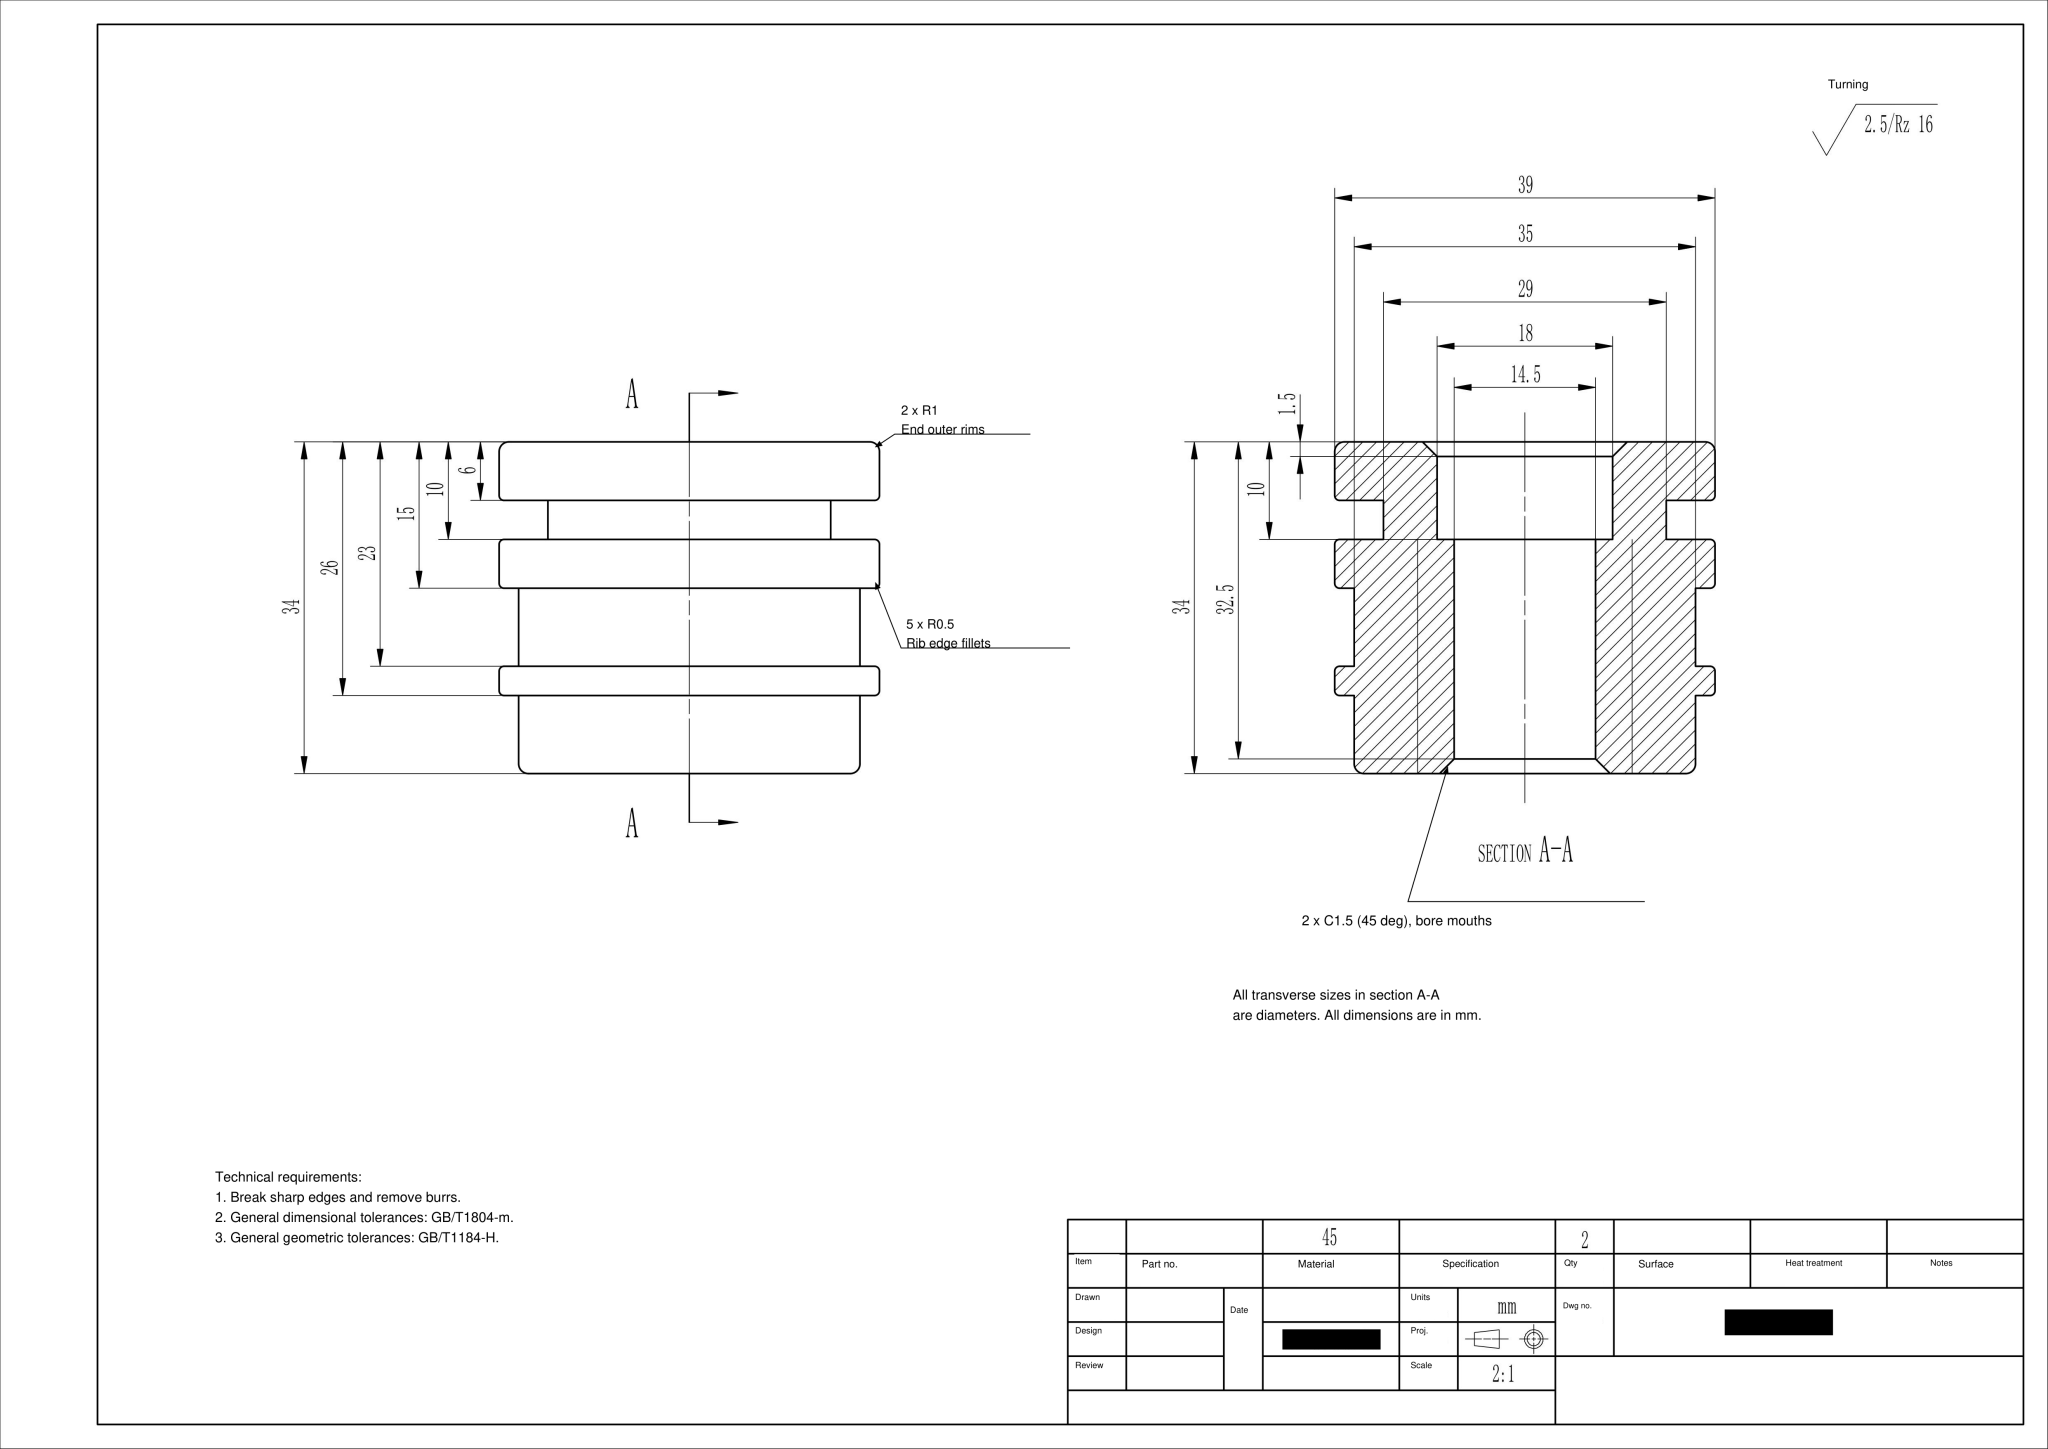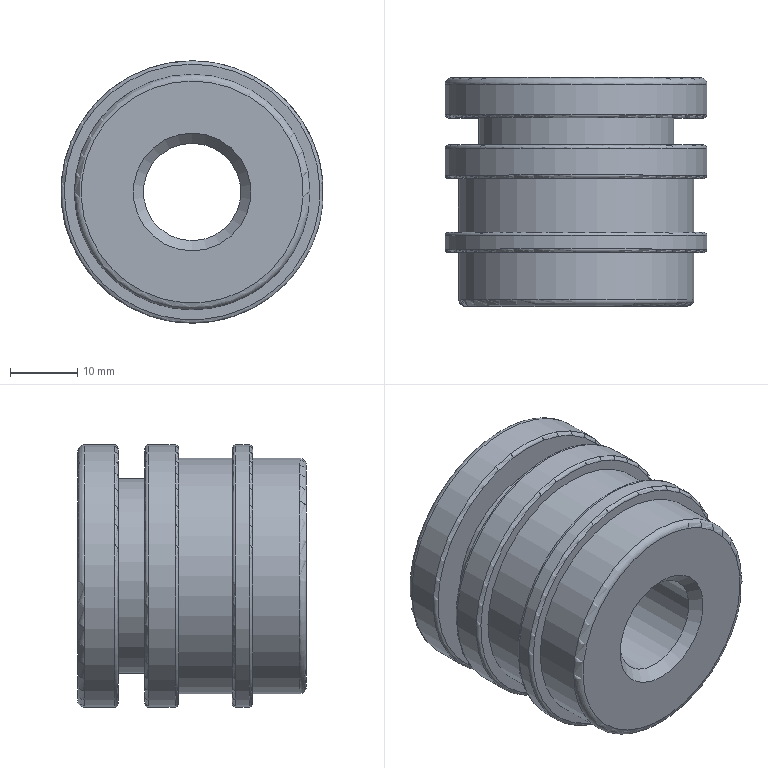Part | NX | mm | 1 solid | 25 faces | box 39 x 34 x 39 mm | volume 28048 mm3 | plane 8 | cylinder 8 | torus 7 | cone 2 | commonest cylinder face diameters 39 x3 35 x2 14.5 x1 18 x1 29 x1
STEP:
#1=CARTESIAN_POINT('',(0.,0.,0.));
#2=DIRECTION('',(0.,0.,1.));
#3=DIRECTION('',(1.,0.,0.));
#4=AXIS2_PLACEMENT_3D('',#1,#2,#3);
#5=(LENGTH_UNIT()NAMED_UNIT(*)SI_UNIT(.MILLI.,.METRE.));
#6=UNCERTAINTY_MEASURE_WITH_UNIT(LENGTH_MEASURE(0.00002),#5,'','');
#7=(NAMED_UNIT(*)PLANE_ANGLE_UNIT()SI_UNIT($,.RADIAN.));
#8=PLANE_ANGLE_MEASURE_WITH_UNIT(PLANE_ANGLE_MEASURE(0.01745),#7);
#9=DIMENSIONAL_EXPONENTS(0.,0.,0.,0.,0.,0.,0.);
#10=(CONVERSION_BASED_UNIT('',#8)NAMED_UNIT(#9)PLANE_ANGLE_UNIT());
#11=(NAMED_UNIT(*)SI_UNIT($,.STERADIAN.)SOLID_ANGLE_UNIT());
#12=(GEOMETRIC_REPRESENTATION_CONTEXT(3)GLOBAL_UNCERTAINTY_ASSIGNED_CONTEXT((#6))GLOBAL_UNIT_ASSIGNED_CONTEXT((#5,#10,#11))REPRESENTATION_CONTEXT('',''));
#13=SHAPE_REPRESENTATION('',(#4),#12);
#14=CARTESIAN_POINT('',(0.,-34.,8.75));
#15=VERTEX_POINT('',#14);
#16=CARTESIAN_POINT('',(0.,-34.,0.));
#17=DIRECTION('',(0.,1.,0.));
#18=DIRECTION('',(0.,0.,1.));
#19=AXIS2_PLACEMENT_3D('',#16,#17,#18);
#20=CIRCLE('',#19,8.75);
#21=EDGE_CURVE('',#15,#15,#20,.T.);
#22=ORIENTED_EDGE('',*,*,#21,.T.);
#23=EDGE_LOOP('',(#22));
#24=FACE_BOUND('',#23,.T.);
#25=CARTESIAN_POINT('',(0.,-34.,16.5));
#26=VERTEX_POINT('',#25);
#27=CARTESIAN_POINT('',(0.,-34.,0.));
#28=DIRECTION('',(0.,-1.,0.));
#29=DIRECTION('',(0.,0.,1.));
#30=AXIS2_PLACEMENT_3D('',#27,#28,#29);
#31=CIRCLE('',#30,16.5);
#32=EDGE_CURVE('',#26,#26,#31,.T.);
#33=ORIENTED_EDGE('',*,*,#32,.T.);
#34=EDGE_LOOP('',(#33));
#35=FACE_BOUND('',#34,.T.);
#36=CARTESIAN_POINT('',(0.,-34.,17.5));
#37=DIRECTION('',(0.,1.,0.));
#38=DIRECTION('',(0.,0.,1.));
#39=AXIS2_PLACEMENT_3D('',#36,#37,#38);
#40=PLANE('',#39);
#41=ADVANCED_FACE('',(#24,#35),#40,.F.);
#42=CARTESIAN_POINT('',(0.,-32.5,7.25));
#43=VERTEX_POINT('',#42);
#44=CARTESIAN_POINT('',(0.,-32.5,0.));
#45=DIRECTION('',(0.,-1.,0.));
#46=DIRECTION('',(0.,0.,1.));
#47=AXIS2_PLACEMENT_3D('',#44,#45,#46);
#48=CIRCLE('',#47,7.25);
#49=EDGE_CURVE('',#43,#43,#48,.T.);
#50=ORIENTED_EDGE('',*,*,#49,.T.);
#51=EDGE_LOOP('',(#50));
#52=FACE_BOUND('',#51,.T.);
#53=CARTESIAN_POINT('',(0.,-10.,-7.25));
#54=VERTEX_POINT('',#53);
#55=CARTESIAN_POINT('',(0.,-10.,0.));
#56=DIRECTION('',(0.,-1.,0.));
#57=DIRECTION('',(0.,0.,-1.));
#58=AXIS2_PLACEMENT_3D('',#55,#56,#57);
#59=CIRCLE('',#58,7.25);
#60=EDGE_CURVE('',#54,#54,#59,.T.);
#61=ORIENTED_EDGE('',*,*,#60,.F.);
#62=EDGE_LOOP('',(#61));
#63=FACE_BOUND('',#62,.T.);
#64=CARTESIAN_POINT('',(0.,0.,0.));
#65=DIRECTION('',(0.,-1.,0.));
#66=DIRECTION('',(0.,0.,-1.));
#67=AXIS2_PLACEMENT_3D('',#64,#65,#66);
#68=CYLINDRICAL_SURFACE('',#67,7.25);
#69=ADVANCED_FACE('',(#52,#63),#68,.F.);
#70=CARTESIAN_POINT('',(0.,-10.,-9.));
#71=VERTEX_POINT('',#70);
#72=CARTESIAN_POINT('',(0.,-10.,0.));
#73=DIRECTION('',(0.,-1.,0.));
#74=DIRECTION('',(0.,0.,-1.));
#75=AXIS2_PLACEMENT_3D('',#72,#73,#74);
#76=CIRCLE('',#75,9.);
#77=EDGE_CURVE('',#71,#71,#76,.T.);
#78=ORIENTED_EDGE('',*,*,#77,.F.);
#79=EDGE_LOOP('',(#78));
#80=FACE_BOUND('',#79,.T.);
#81=ORIENTED_EDGE('',*,*,#60,.T.);
#82=EDGE_LOOP('',(#81));
#83=FACE_BOUND('',#82,.T.);
#84=CARTESIAN_POINT('',(0.,-10.,7.25));
#85=DIRECTION('',(0.,-1.,0.));
#86=DIRECTION('',(0.,0.,-1.));
#87=AXIS2_PLACEMENT_3D('',#84,#85,#86);
#88=PLANE('',#87);
#89=ADVANCED_FACE('',(#80,#83),#88,.F.);
#90=CARTESIAN_POINT('',(0.,-1.5,-9.));
#91=VERTEX_POINT('',#90);
#92=CARTESIAN_POINT('',(0.,-1.5,0.));
#93=DIRECTION('',(0.,1.,0.));
#94=DIRECTION('',(0.,0.,-1.));
#95=AXIS2_PLACEMENT_3D('',#92,#93,#94);
#96=CIRCLE('',#95,9.);
#97=EDGE_CURVE('',#91,#91,#96,.T.);
#98=ORIENTED_EDGE('',*,*,#97,.T.);
#99=EDGE_LOOP('',(#98));
#100=FACE_BOUND('',#99,.T.);
#101=ORIENTED_EDGE('',*,*,#77,.T.);
#102=EDGE_LOOP('',(#101));
#103=FACE_BOUND('',#102,.T.);
#104=CARTESIAN_POINT('',(0.,0.,0.));
#105=DIRECTION('',(0.,-1.,0.));
#106=DIRECTION('',(0.,0.,-1.));
#107=AXIS2_PLACEMENT_3D('',#104,#105,#106);
#108=CYLINDRICAL_SURFACE('',#107,9.);
#109=ADVANCED_FACE('',(#100,#103),#108,.F.);
#110=CARTESIAN_POINT('',(0.,0.,-10.5));
#111=VERTEX_POINT('',#110);
#112=CARTESIAN_POINT('',(0.,0.,0.));
#113=DIRECTION('',(0.,-1.,0.));
#114=DIRECTION('',(0.,0.,-1.));
#115=AXIS2_PLACEMENT_3D('',#112,#113,#114);
#116=CIRCLE('',#115,10.5);
#117=EDGE_CURVE('',#111,#111,#116,.T.);
#118=ORIENTED_EDGE('',*,*,#117,.T.);
#119=EDGE_LOOP('',(#118));
#120=FACE_BOUND('',#119,.T.);
#121=CARTESIAN_POINT('',(0.,0.,-18.5));
#122=VERTEX_POINT('',#121);
#123=CARTESIAN_POINT('',(0.,0.,0.));
#124=DIRECTION('',(0.,1.,0.));
#125=DIRECTION('',(0.,0.,-1.));
#126=AXIS2_PLACEMENT_3D('',#123,#124,#125);
#127=CIRCLE('',#126,18.5);
#128=EDGE_CURVE('',#122,#122,#127,.T.);
#129=ORIENTED_EDGE('',*,*,#128,.T.);
#130=EDGE_LOOP('',(#129));
#131=FACE_BOUND('',#130,.T.);
#132=CARTESIAN_POINT('',(0.,0.,9.));
#133=DIRECTION('',(0.,-1.,0.));
#134=DIRECTION('',(0.,0.,-1.));
#135=AXIS2_PLACEMENT_3D('',#132,#133,#134);
#136=PLANE('',#135);
#137=ADVANCED_FACE('',(#120,#131),#136,.F.);
#138=CARTESIAN_POINT('',(0.,-5.5,19.5));
#139=VERTEX_POINT('',#138);
#140=CARTESIAN_POINT('',(0.,-5.5,0.));
#141=DIRECTION('',(0.,1.,0.));
#142=DIRECTION('',(0.,0.,1.));
#143=AXIS2_PLACEMENT_3D('',#140,#141,#142);
#144=CIRCLE('',#143,19.5);
#145=EDGE_CURVE('',#139,#139,#144,.T.);
#146=ORIENTED_EDGE('',*,*,#145,.T.);
#147=EDGE_LOOP('',(#146));
#148=FACE_BOUND('',#147,.T.);
#149=CARTESIAN_POINT('',(0.,-1.,-19.5));
#150=VERTEX_POINT('',#149);
#151=CARTESIAN_POINT('',(0.,-1.,0.));
#152=DIRECTION('',(0.,-1.,0.));
#153=DIRECTION('',(0.,0.,-1.));
#154=AXIS2_PLACEMENT_3D('',#151,#152,#153);
#155=CIRCLE('',#154,19.5);
#156=EDGE_CURVE('',#150,#150,#155,.T.);
#157=ORIENTED_EDGE('',*,*,#156,.T.);
#158=EDGE_LOOP('',(#157));
#159=FACE_BOUND('',#158,.T.);
#160=CARTESIAN_POINT('',(0.,0.,0.));
#161=DIRECTION('',(0.,-1.,0.));
#162=DIRECTION('',(0.,0.,-1.));
#163=AXIS2_PLACEMENT_3D('',#160,#161,#162);
#164=CYLINDRICAL_SURFACE('',#163,19.5);
#165=ADVANCED_FACE('',(#148,#159),#164,.T.);
#166=CARTESIAN_POINT('',(0.,-6.,19.));
#167=VERTEX_POINT('',#166);
#168=CARTESIAN_POINT('',(0.,-6.,0.));
#169=DIRECTION('',(0.,-1.,0.));
#170=DIRECTION('',(0.,0.,1.));
#171=AXIS2_PLACEMENT_3D('',#168,#169,#170);
#172=CIRCLE('',#171,19.);
#173=EDGE_CURVE('',#167,#167,#172,.T.);
#174=ORIENTED_EDGE('',*,*,#173,.T.);
#175=EDGE_LOOP('',(#174));
#176=FACE_BOUND('',#175,.T.);
#177=CARTESIAN_POINT('',(0.,-6.,-14.5));
#178=VERTEX_POINT('',#177);
#179=CARTESIAN_POINT('',(0.,-6.,0.));
#180=DIRECTION('',(0.,-1.,0.));
#181=DIRECTION('',(0.,0.,-1.));
#182=AXIS2_PLACEMENT_3D('',#179,#180,#181);
#183=CIRCLE('',#182,14.5);
#184=EDGE_CURVE('',#178,#178,#183,.T.);
#185=ORIENTED_EDGE('',*,*,#184,.F.);
#186=EDGE_LOOP('',(#185));
#187=FACE_BOUND('',#186,.T.);
#188=CARTESIAN_POINT('',(0.,-6.,19.5));
#189=DIRECTION('',(0.,1.,0.));
#190=DIRECTION('',(0.,0.,1.));
#191=AXIS2_PLACEMENT_3D('',#188,#189,#190);
#192=PLANE('',#191);
#193=ADVANCED_FACE('',(#176,#187),#192,.F.);
#194=CARTESIAN_POINT('',(0.,-10.,-14.5));
#195=VERTEX_POINT('',#194);
#196=CARTESIAN_POINT('',(0.,-10.,0.));
#197=DIRECTION('',(0.,-1.,0.));
#198=DIRECTION('',(0.,0.,-1.));
#199=AXIS2_PLACEMENT_3D('',#196,#197,#198);
#200=CIRCLE('',#199,14.5);
#201=EDGE_CURVE('',#195,#195,#200,.T.);
#202=ORIENTED_EDGE('',*,*,#201,.F.);
#203=EDGE_LOOP('',(#202));
#204=FACE_BOUND('',#203,.T.);
#205=ORIENTED_EDGE('',*,*,#184,.T.);
#206=EDGE_LOOP('',(#205));
#207=FACE_BOUND('',#206,.T.);
#208=CARTESIAN_POINT('',(0.,0.,0.));
#209=DIRECTION('',(0.,-1.,0.));
#210=DIRECTION('',(0.,0.,-1.));
#211=AXIS2_PLACEMENT_3D('',#208,#209,#210);
#212=CYLINDRICAL_SURFACE('',#211,14.5);
#213=ADVANCED_FACE('',(#204,#207),#212,.T.);
#214=CARTESIAN_POINT('',(0.,-10.,-19.));
#215=VERTEX_POINT('',#214);
#216=CARTESIAN_POINT('',(0.,-10.,0.));
#217=DIRECTION('',(0.,1.,0.));
#218=DIRECTION('',(0.,0.,-1.));
#219=AXIS2_PLACEMENT_3D('',#216,#217,#218);
#220=CIRCLE('',#219,19.);
#221=EDGE_CURVE('',#215,#215,#220,.T.);
#222=ORIENTED_EDGE('',*,*,#221,.T.);
#223=EDGE_LOOP('',(#222));
#224=FACE_BOUND('',#223,.T.);
#225=ORIENTED_EDGE('',*,*,#201,.T.);
#226=EDGE_LOOP('',(#225));
#227=FACE_BOUND('',#226,.T.);
#228=CARTESIAN_POINT('',(0.,-10.,14.5));
#229=DIRECTION('',(0.,-1.,0.));
#230=DIRECTION('',(0.,0.,-1.));
#231=AXIS2_PLACEMENT_3D('',#228,#229,#230);
#232=PLANE('',#231);
#233=ADVANCED_FACE('',(#224,#227),#232,.F.);
#234=CARTESIAN_POINT('',(0.,-14.5,19.5));
#235=VERTEX_POINT('',#234);
#236=CARTESIAN_POINT('',(0.,-14.5,0.));
#237=DIRECTION('',(0.,1.,0.));
#238=DIRECTION('',(0.,0.,1.));
#239=AXIS2_PLACEMENT_3D('',#236,#237,#238);
#240=CIRCLE('',#239,19.5);
#241=EDGE_CURVE('',#235,#235,#240,.T.);
#242=ORIENTED_EDGE('',*,*,#241,.T.);
#243=EDGE_LOOP('',(#242));
#244=FACE_BOUND('',#243,.T.);
#245=CARTESIAN_POINT('',(0.,-10.5,-19.5));
#246=VERTEX_POINT('',#245);
#247=CARTESIAN_POINT('',(0.,-10.5,0.));
#248=DIRECTION('',(0.,-1.,0.));
#249=DIRECTION('',(0.,0.,-1.));
#250=AXIS2_PLACEMENT_3D('',#247,#248,#249);
#251=CIRCLE('',#250,19.5);
#252=EDGE_CURVE('',#246,#246,#251,.T.);
#253=ORIENTED_EDGE('',*,*,#252,.T.);
#254=EDGE_LOOP('',(#253));
#255=FACE_BOUND('',#254,.T.);
#256=CARTESIAN_POINT('',(0.,0.,0.));
#257=DIRECTION('',(0.,-1.,0.));
#258=DIRECTION('',(0.,0.,-1.));
#259=AXIS2_PLACEMENT_3D('',#256,#257,#258);
#260=CYLINDRICAL_SURFACE('',#259,19.5);
#261=ADVANCED_FACE('',(#244,#255),#260,.T.);
#262=CARTESIAN_POINT('',(0.,-15.,19.));
#263=VERTEX_POINT('',#262);
#264=CARTESIAN_POINT('',(0.,-15.,0.));
#265=DIRECTION('',(0.,-1.,0.));
#266=DIRECTION('',(0.,0.,1.));
#267=AXIS2_PLACEMENT_3D('',#264,#265,#266);
#268=CIRCLE('',#267,19.);
#269=EDGE_CURVE('',#263,#263,#268,.T.);
#270=ORIENTED_EDGE('',*,*,#269,.T.);
#271=EDGE_LOOP('',(#270));
#272=FACE_BOUND('',#271,.T.);
#273=CARTESIAN_POINT('',(0.,-15.,-17.5));
#274=VERTEX_POINT('',#273);
#275=CARTESIAN_POINT('',(0.,-15.,0.));
#276=DIRECTION('',(0.,-1.,0.));
#277=DIRECTION('',(0.,0.,-1.));
#278=AXIS2_PLACEMENT_3D('',#275,#276,#277);
#279=CIRCLE('',#278,17.5);
#280=EDGE_CURVE('',#274,#274,#279,.T.);
#281=ORIENTED_EDGE('',*,*,#280,.F.);
#282=EDGE_LOOP('',(#281));
#283=FACE_BOUND('',#282,.T.);
#284=CARTESIAN_POINT('',(0.,-15.,19.5));
#285=DIRECTION('',(0.,1.,0.));
#286=DIRECTION('',(0.,0.,1.));
#287=AXIS2_PLACEMENT_3D('',#284,#285,#286);
#288=PLANE('',#287);
#289=ADVANCED_FACE('',(#272,#283),#288,.F.);
#290=CARTESIAN_POINT('',(0.,-23.,-17.5));
#291=VERTEX_POINT('',#290);
#292=CARTESIAN_POINT('',(0.,-23.,0.));
#293=DIRECTION('',(0.,-1.,0.));
#294=DIRECTION('',(0.,0.,-1.));
#295=AXIS2_PLACEMENT_3D('',#292,#293,#294);
#296=CIRCLE('',#295,17.5);
#297=EDGE_CURVE('',#291,#291,#296,.T.);
#298=ORIENTED_EDGE('',*,*,#297,.F.);
#299=EDGE_LOOP('',(#298));
#300=FACE_BOUND('',#299,.T.);
#301=ORIENTED_EDGE('',*,*,#280,.T.);
#302=EDGE_LOOP('',(#301));
#303=FACE_BOUND('',#302,.T.);
#304=CARTESIAN_POINT('',(0.,0.,0.));
#305=DIRECTION('',(0.,-1.,0.));
#306=DIRECTION('',(0.,0.,-1.));
#307=AXIS2_PLACEMENT_3D('',#304,#305,#306);
#308=CYLINDRICAL_SURFACE('',#307,17.5);
#309=ADVANCED_FACE('',(#300,#303),#308,.T.);
#310=CARTESIAN_POINT('',(0.,-23.,-19.));
#311=VERTEX_POINT('',#310);
#312=CARTESIAN_POINT('',(0.,-23.,0.));
#313=DIRECTION('',(0.,1.,0.));
#314=DIRECTION('',(0.,0.,-1.));
#315=AXIS2_PLACEMENT_3D('',#312,#313,#314);
#316=CIRCLE('',#315,19.);
#317=EDGE_CURVE('',#311,#311,#316,.T.);
#318=ORIENTED_EDGE('',*,*,#317,.T.);
#319=EDGE_LOOP('',(#318));
#320=FACE_BOUND('',#319,.T.);
#321=ORIENTED_EDGE('',*,*,#297,.T.);
#322=EDGE_LOOP('',(#321));
#323=FACE_BOUND('',#322,.T.);
#324=CARTESIAN_POINT('',(0.,-23.,17.5));
#325=DIRECTION('',(0.,-1.,0.));
#326=DIRECTION('',(0.,0.,-1.));
#327=AXIS2_PLACEMENT_3D('',#324,#325,#326);
#328=PLANE('',#327);
#329=ADVANCED_FACE('',(#320,#323),#328,.F.);
#330=CARTESIAN_POINT('',(0.,-25.5,19.5));
#331=VERTEX_POINT('',#330);
#332=CARTESIAN_POINT('',(0.,-25.5,0.));
#333=DIRECTION('',(0.,1.,0.));
#334=DIRECTION('',(0.,0.,1.));
#335=AXIS2_PLACEMENT_3D('',#332,#333,#334);
#336=CIRCLE('',#335,19.5);
#337=EDGE_CURVE('',#331,#331,#336,.T.);
#338=ORIENTED_EDGE('',*,*,#337,.T.);
#339=EDGE_LOOP('',(#338));
#340=FACE_BOUND('',#339,.T.);
#341=CARTESIAN_POINT('',(0.,-23.5,-19.5));
#342=VERTEX_POINT('',#341);
#343=CARTESIAN_POINT('',(0.,-23.5,0.));
#344=DIRECTION('',(0.,-1.,0.));
#345=DIRECTION('',(0.,0.,-1.));
#346=AXIS2_PLACEMENT_3D('',#343,#344,#345);
#347=CIRCLE('',#346,19.5);
#348=EDGE_CURVE('',#342,#342,#347,.T.);
#349=ORIENTED_EDGE('',*,*,#348,.T.);
#350=EDGE_LOOP('',(#349));
#351=FACE_BOUND('',#350,.T.);
#352=CARTESIAN_POINT('',(0.,0.,0.));
#353=DIRECTION('',(0.,-1.,0.));
#354=DIRECTION('',(0.,0.,-1.));
#355=AXIS2_PLACEMENT_3D('',#352,#353,#354);
#356=CYLINDRICAL_SURFACE('',#355,19.5);
#357=ADVANCED_FACE('',(#340,#351),#356,.T.);
#358=CARTESIAN_POINT('',(0.,-26.,19.));
#359=VERTEX_POINT('',#358);
#360=CARTESIAN_POINT('',(0.,-26.,0.));
#361=DIRECTION('',(0.,-1.,0.));
#362=DIRECTION('',(0.,0.,1.));
#363=AXIS2_PLACEMENT_3D('',#360,#361,#362);
#364=CIRCLE('',#363,19.);
#365=EDGE_CURVE('',#359,#359,#364,.T.);
#366=ORIENTED_EDGE('',*,*,#365,.T.);
#367=EDGE_LOOP('',(#366));
#368=FACE_BOUND('',#367,.T.);
#369=CARTESIAN_POINT('',(0.,-26.,-17.5));
#370=VERTEX_POINT('',#369);
#371=CARTESIAN_POINT('',(0.,-26.,0.));
#372=DIRECTION('',(0.,-1.,0.));
#373=DIRECTION('',(0.,0.,-1.));
#374=AXIS2_PLACEMENT_3D('',#371,#372,#373);
#375=CIRCLE('',#374,17.5);
#376=EDGE_CURVE('',#370,#370,#375,.T.);
#377=ORIENTED_EDGE('',*,*,#376,.F.);
#378=EDGE_LOOP('',(#377));
#379=FACE_BOUND('',#378,.T.);
#380=CARTESIAN_POINT('',(0.,-26.,19.5));
#381=DIRECTION('',(0.,1.,0.));
#382=DIRECTION('',(0.,0.,1.));
#383=AXIS2_PLACEMENT_3D('',#380,#381,#382);
#384=PLANE('',#383);
#385=ADVANCED_FACE('',(#368,#379),#384,.F.);
#386=CARTESIAN_POINT('',(0.,-33.,17.5));
#387=VERTEX_POINT('',#386);
#388=CARTESIAN_POINT('',(0.,-33.,0.));
#389=DIRECTION('',(0.,1.,0.));
#390=DIRECTION('',(0.,0.,1.));
#391=AXIS2_PLACEMENT_3D('',#388,#389,#390);
#392=CIRCLE('',#391,17.5);
#393=EDGE_CURVE('',#387,#387,#392,.T.);
#394=ORIENTED_EDGE('',*,*,#393,.T.);
#395=EDGE_LOOP('',(#394));
#396=FACE_BOUND('',#395,.T.);
#397=ORIENTED_EDGE('',*,*,#376,.T.);
#398=EDGE_LOOP('',(#397));
#399=FACE_BOUND('',#398,.T.);
#400=CARTESIAN_POINT('',(0.,0.,0.));
#401=DIRECTION('',(0.,-1.,0.));
#402=DIRECTION('',(0.,0.,-1.));
#403=AXIS2_PLACEMENT_3D('',#400,#401,#402);
#404=CYLINDRICAL_SURFACE('',#403,17.5);
#405=ADVANCED_FACE('',(#396,#399),#404,.T.);
#406=ORIENTED_EDGE('',*,*,#393,.F.);
#407=EDGE_LOOP('',(#406));
#408=FACE_BOUND('',#407,.T.);
#409=ORIENTED_EDGE('',*,*,#32,.F.);
#410=EDGE_LOOP('',(#409));
#411=FACE_BOUND('',#410,.T.);
#412=CARTESIAN_POINT('',(0.,-33.,0.));
#413=DIRECTION('',(0.,1.,0.));
#414=DIRECTION('',(0.,0.,1.));
#415=AXIS2_PLACEMENT_3D('',#412,#413,#414);
#416=TOROIDAL_SURFACE('',#415,16.5,1.);
#417=ADVANCED_FACE('',(#408,#411),#416,.T.);
#418=ORIENTED_EDGE('',*,*,#128,.F.);
#419=EDGE_LOOP('',(#418));
#420=FACE_BOUND('',#419,.T.);
#421=ORIENTED_EDGE('',*,*,#156,.F.);
#422=EDGE_LOOP('',(#421));
#423=FACE_BOUND('',#422,.T.);
#424=CARTESIAN_POINT('',(0.,-1.,0.));
#425=DIRECTION('',(0.,-1.,0.));
#426=DIRECTION('',(0.,0.,-1.));
#427=AXIS2_PLACEMENT_3D('',#424,#425,#426);
#428=TOROIDAL_SURFACE('',#427,18.5,1.);
#429=ADVANCED_FACE('',(#420,#423),#428,.T.);
#430=ORIENTED_EDGE('',*,*,#337,.F.);
#431=EDGE_LOOP('',(#430));
#432=FACE_BOUND('',#431,.T.);
#433=ORIENTED_EDGE('',*,*,#365,.F.);
#434=EDGE_LOOP('',(#433));
#435=FACE_BOUND('',#434,.T.);
#436=CARTESIAN_POINT('',(0.,-25.5,0.));
#437=DIRECTION('',(0.,1.,0.));
#438=DIRECTION('',(0.,0.,1.));
#439=AXIS2_PLACEMENT_3D('',#436,#437,#438);
#440=TOROIDAL_SURFACE('',#439,19.,0.5);
#441=ADVANCED_FACE('',(#432,#435),#440,.T.);
#442=ORIENTED_EDGE('',*,*,#317,.F.);
#443=EDGE_LOOP('',(#442));
#444=FACE_BOUND('',#443,.T.);
#445=ORIENTED_EDGE('',*,*,#348,.F.);
#446=EDGE_LOOP('',(#445));
#447=FACE_BOUND('',#446,.T.);
#448=CARTESIAN_POINT('',(0.,-23.5,0.));
#449=DIRECTION('',(0.,-1.,0.));
#450=DIRECTION('',(0.,0.,-1.));
#451=AXIS2_PLACEMENT_3D('',#448,#449,#450);
#452=TOROIDAL_SURFACE('',#451,19.,0.5);
#453=ADVANCED_FACE('',(#444,#447),#452,.T.);
#454=ORIENTED_EDGE('',*,*,#241,.F.);
#455=EDGE_LOOP('',(#454));
#456=FACE_BOUND('',#455,.T.);
#457=ORIENTED_EDGE('',*,*,#269,.F.);
#458=EDGE_LOOP('',(#457));
#459=FACE_BOUND('',#458,.T.);
#460=CARTESIAN_POINT('',(0.,-14.5,0.));
#461=DIRECTION('',(0.,1.,0.));
#462=DIRECTION('',(0.,0.,1.));
#463=AXIS2_PLACEMENT_3D('',#460,#461,#462);
#464=TOROIDAL_SURFACE('',#463,19.,0.5);
#465=ADVANCED_FACE('',(#456,#459),#464,.T.);
#466=ORIENTED_EDGE('',*,*,#221,.F.);
#467=EDGE_LOOP('',(#466));
#468=FACE_BOUND('',#467,.T.);
#469=ORIENTED_EDGE('',*,*,#252,.F.);
#470=EDGE_LOOP('',(#469));
#471=FACE_BOUND('',#470,.T.);
#472=CARTESIAN_POINT('',(0.,-10.5,0.));
#473=DIRECTION('',(0.,-1.,0.));
#474=DIRECTION('',(0.,0.,-1.));
#475=AXIS2_PLACEMENT_3D('',#472,#473,#474);
#476=TOROIDAL_SURFACE('',#475,19.,0.5);
#477=ADVANCED_FACE('',(#468,#471),#476,.T.);
#478=ORIENTED_EDGE('',*,*,#145,.F.);
#479=EDGE_LOOP('',(#478));
#480=FACE_BOUND('',#479,.T.);
#481=ORIENTED_EDGE('',*,*,#173,.F.);
#482=EDGE_LOOP('',(#481));
#483=FACE_BOUND('',#482,.T.);
#484=CARTESIAN_POINT('',(0.,-5.5,0.));
#485=DIRECTION('',(0.,1.,0.));
#486=DIRECTION('',(0.,0.,1.));
#487=AXIS2_PLACEMENT_3D('',#484,#485,#486);
#488=TOROIDAL_SURFACE('',#487,19.,0.5);
#489=ADVANCED_FACE('',(#480,#483),#488,.T.);
#490=ORIENTED_EDGE('',*,*,#97,.F.);
#491=EDGE_LOOP('',(#490));
#492=FACE_BOUND('',#491,.T.);
#493=ORIENTED_EDGE('',*,*,#117,.F.);
#494=EDGE_LOOP('',(#493));
#495=FACE_BOUND('',#494,.T.);
#496=CARTESIAN_POINT('',(0.,0.,0.));
#497=DIRECTION('',(0.,1.,0.));
#498=DIRECTION('',(0.,0.,1.));
#499=AXIS2_PLACEMENT_3D('',#496,#497,#498);
#500=CONICAL_SURFACE('',#499,10.5,45.);
#501=ADVANCED_FACE('',(#492,#495),#500,.F.);
#502=ORIENTED_EDGE('',*,*,#21,.F.);
#503=EDGE_LOOP('',(#502));
#504=FACE_BOUND('',#503,.T.);
#505=ORIENTED_EDGE('',*,*,#49,.F.);
#506=EDGE_LOOP('',(#505));
#507=FACE_BOUND('',#506,.T.);
#508=CARTESIAN_POINT('',(0.,-32.5,0.));
#509=DIRECTION('',(0.,-1.,0.));
#510=DIRECTION('',(0.,0.,-1.));
#511=AXIS2_PLACEMENT_3D('',#508,#509,#510);
#512=CONICAL_SURFACE('',#511,7.25,45.);
#513=ADVANCED_FACE('',(#504,#507),#512,.F.);
#514=CLOSED_SHELL('',(#41,#69,#89,#109,#137,#165,#193,#213,#233,#261,#289,#309,#329,#357,#385,#405,#417,#429,#441,#453,#465,#477,#489,#501,#513));
#515=MANIFOLD_SOLID_BREP('',#514);
#516=ADVANCED_BREP_SHAPE_REPRESENTATION('',(#515),#12);
#517=SHAPE_REPRESENTATION_RELATIONSHIP('','',#13,#516);
#518=PRESENTATION_LAYER_ASSIGNMENT('','',(#515));
#519=COLOUR_RGB('',0.6118,0.6588,0.6706);
#520=FILL_AREA_STYLE_COLOUR('',#519);
#521=FILL_AREA_STYLE('',(#520));
#522=SURFACE_STYLE_FILL_AREA(#521);
#523=SURFACE_SIDE_STYLE('',(#522));
#524=SURFACE_STYLE_USAGE(.BOTH.,#523);
#525=PRESENTATION_STYLE_ASSIGNMENT((#524));
#526=STYLED_ITEM('',(#525),#515);
#527=MECHANICAL_DESIGN_GEOMETRIC_PRESENTATION_REPRESENTATION('',(#526),#12);